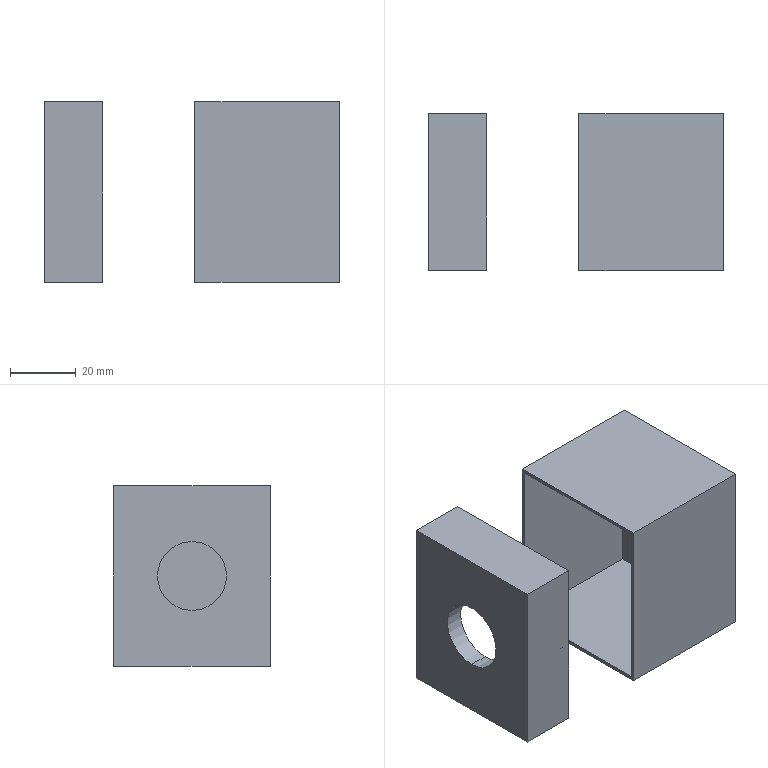Component | SolidWorks | BearingHousing-1 | 2 solids | 29 faces | box 89.77 x 47.79 x 55 mm | volume 29257 mm3 | plane 24 | cylinder 5 | commonest cylinder face diameters 47.04 x3 21 x2
STEP:
#1=COLOUR_RGB('',0.7922,0.8196,0.9333);
#2=FILL_AREA_STYLE_COLOUR('',#1);
#3=FILL_AREA_STYLE('',(#2));
#4=SURFACE_STYLE_FILL_AREA(#3);
#5=SURFACE_SIDE_STYLE('',(#4));
#6=SURFACE_STYLE_USAGE(.BOTH.,#5);
#7=PRESENTATION_STYLE_ASSIGNMENT((#6));
#8=CARTESIAN_POINT('',(7.039,3.272,1.043));
#9=VERTEX_POINT('',#8);
#10=CARTESIAN_POINT('',(7.039,1.469,1.043));
#11=VERTEX_POINT('',#10);
#12=CARTESIAN_POINT('',(7.039,3.37,1.043));
#13=DIRECTION('',(0.,-1.,0.));
#14=VECTOR('',#13,39.37);
#15=LINE('',#12,#14);
#16=EDGE_CURVE('',#9,#11,#15,.T.);
#17=ORIENTED_EDGE('',*,*,#16,.T.);
#18=CARTESIAN_POINT('',(7.039,1.469,-1.043));
#19=VERTEX_POINT('',#18);
#20=CARTESIAN_POINT('',(7.039,1.469,0.8331));
#21=DIRECTION('',(-0.,-0.,-1.));
#22=VECTOR('',#21,39.37);
#23=LINE('',#20,#22);
#24=EDGE_CURVE('',#11,#19,#23,.T.);
#25=ORIENTED_EDGE('',*,*,#24,.T.);
#26=CARTESIAN_POINT('',(7.039,3.272,-1.043));
#27=VERTEX_POINT('',#26);
#28=CARTESIAN_POINT('',(7.039,3.37,-1.043));
#29=DIRECTION('',(-0.,1.,-0.));
#30=VECTOR('',#29,39.37);
#31=LINE('',#28,#30);
#32=EDGE_CURVE('',#19,#27,#31,.T.);
#33=ORIENTED_EDGE('',*,*,#32,.T.);
#34=CARTESIAN_POINT('',(7.039,3.272,0.8331));
#35=DIRECTION('',(0.,0.,1.));
#36=VECTOR('',#35,39.37);
#37=LINE('',#34,#36);
#38=EDGE_CURVE('',#27,#9,#37,.T.);
#39=ORIENTED_EDGE('',*,*,#38,.T.);
#40=EDGE_LOOP('',(#17,#25,#33,#39));
#41=FACE_BOUND('',#40,.T.);
#42=CARTESIAN_POINT('',(7.039,1.43,1.083));
#43=VERTEX_POINT('',#42);
#44=CARTESIAN_POINT('',(7.039,1.43,-1.083));
#45=VERTEX_POINT('',#44);
#46=CARTESIAN_POINT('',(7.039,1.43,1.083));
#47=DIRECTION('',(-0.,-0.,-1.));
#48=VECTOR('',#47,39.37);
#49=LINE('',#46,#48);
#50=EDGE_CURVE('',#43,#45,#49,.T.);
#51=ORIENTED_EDGE('',*,*,#50,.F.);
#52=CARTESIAN_POINT('',(7.039,3.312,1.083));
#53=VERTEX_POINT('',#52);
#54=CARTESIAN_POINT('',(7.039,3.312,1.083));
#55=DIRECTION('',(0.,-1.,0.));
#56=VECTOR('',#55,39.37);
#57=LINE('',#54,#56);
#58=EDGE_CURVE('',#53,#43,#57,.T.);
#59=ORIENTED_EDGE('',*,*,#58,.F.);
#60=CARTESIAN_POINT('',(7.039,3.312,-1.083));
#61=VERTEX_POINT('',#60);
#62=CARTESIAN_POINT('',(7.039,3.312,-1.083));
#63=DIRECTION('',(0.,0.,1.));
#64=VECTOR('',#63,39.37);
#65=LINE('',#62,#64);
#66=EDGE_CURVE('',#61,#53,#65,.T.);
#67=ORIENTED_EDGE('',*,*,#66,.F.);
#68=CARTESIAN_POINT('',(7.039,1.43,-1.083));
#69=DIRECTION('',(-0.,1.,-0.));
#70=VECTOR('',#69,39.37);
#71=LINE('',#68,#70);
#72=EDGE_CURVE('',#45,#61,#71,.T.);
#73=ORIENTED_EDGE('',*,*,#72,.F.);
#74=EDGE_LOOP('',(#51,#59,#67,#73));
#75=FACE_OUTER_BOUND('',#74,.T.);
#76=CARTESIAN_POINT('',(7.039,3.37,0.8331));
#77=DIRECTION('',(1.,0.,-0.));
#78=DIRECTION('',(0.,-1.,0.));
#79=AXIS2_PLACEMENT_3D('',#76,#77,#78);
#80=PLANE('',#79);
#81=ADVANCED_FACE('',(#41,#75),#80,.F.);
#82=CARTESIAN_POINT('',(8.771,1.43,-1.083));
#83=VERTEX_POINT('',#82);
#84=CARTESIAN_POINT('',(-2.164,1.43,-1.083));
#85=DIRECTION('',(1.,-0.,0.));
#86=VECTOR('',#85,39.37);
#87=LINE('',#84,#86);
#88=EDGE_CURVE('',#45,#83,#87,.T.);
#89=ORIENTED_EDGE('',*,*,#88,.F.);
#90=ORIENTED_EDGE('',*,*,#72,.T.);
#91=CARTESIAN_POINT('',(8.771,3.312,-1.083));
#92=VERTEX_POINT('',#91);
#93=CARTESIAN_POINT('',(-2.164,3.312,-1.083));
#94=DIRECTION('',(-1.,-0.,-0.));
#95=VECTOR('',#94,39.37);
#96=LINE('',#93,#95);
#97=EDGE_CURVE('',#92,#61,#96,.T.);
#98=ORIENTED_EDGE('',*,*,#97,.F.);
#99=CARTESIAN_POINT('',(8.771,1.43,-1.083));
#100=DIRECTION('',(-0.,1.,-0.));
#101=VECTOR('',#100,39.37);
#102=LINE('',#99,#101);
#103=EDGE_CURVE('',#83,#92,#102,.T.);
#104=ORIENTED_EDGE('',*,*,#103,.F.);
#105=EDGE_LOOP('',(#89,#90,#98,#104));
#106=FACE_OUTER_BOUND('',#105,.T.);
#107=CARTESIAN_POINT('',(-2.164,3.37,-1.083));
#108=DIRECTION('',(-0.,0.,1.));
#109=DIRECTION('',(0.,-1.,0.));
#110=AXIS2_PLACEMENT_3D('',#107,#108,#109);
#111=PLANE('',#110);
#112=ADVANCED_FACE('',(#106),#111,.F.);
#113=ORIENTED_EDGE('',*,*,#58,.T.);
#114=CARTESIAN_POINT('',(8.771,1.43,1.083));
#115=VERTEX_POINT('',#114);
#116=CARTESIAN_POINT('',(-2.164,1.43,1.083));
#117=DIRECTION('',(1.,-0.,0.));
#118=VECTOR('',#117,39.37);
#119=LINE('',#116,#118);
#120=EDGE_CURVE('',#43,#115,#119,.T.);
#121=ORIENTED_EDGE('',*,*,#120,.T.);
#122=CARTESIAN_POINT('',(8.771,3.312,1.083));
#123=VERTEX_POINT('',#122);
#124=CARTESIAN_POINT('',(8.771,3.312,1.083));
#125=DIRECTION('',(0.,-1.,0.));
#126=VECTOR('',#125,39.37);
#127=LINE('',#124,#126);
#128=EDGE_CURVE('',#123,#115,#127,.T.);
#129=ORIENTED_EDGE('',*,*,#128,.F.);
#130=CARTESIAN_POINT('',(-2.164,3.312,1.083));
#131=DIRECTION('',(-1.,-0.,-0.));
#132=VECTOR('',#131,39.37);
#133=LINE('',#130,#132);
#134=EDGE_CURVE('',#123,#53,#133,.T.);
#135=ORIENTED_EDGE('',*,*,#134,.T.);
#136=EDGE_LOOP('',(#113,#121,#129,#135));
#137=FACE_OUTER_BOUND('',#136,.T.);
#138=CARTESIAN_POINT('',(-2.164,3.37,1.083));
#139=DIRECTION('',(-0.,0.,1.));
#140=DIRECTION('',(0.,-1.,0.));
#141=AXIS2_PLACEMENT_3D('',#138,#139,#140);
#142=PLANE('',#141);
#143=ADVANCED_FACE('',(#137),#142,.T.);
#144=ORIENTED_EDGE('',*,*,#120,.F.);
#145=ORIENTED_EDGE('',*,*,#50,.T.);
#146=ORIENTED_EDGE('',*,*,#88,.T.);
#147=CARTESIAN_POINT('',(8.771,1.43,1.083));
#148=DIRECTION('',(-0.,-0.,-1.));
#149=VECTOR('',#148,39.37);
#150=LINE('',#147,#149);
#151=EDGE_CURVE('',#115,#83,#150,.T.);
#152=ORIENTED_EDGE('',*,*,#151,.F.);
#153=EDGE_LOOP('',(#144,#145,#146,#152));
#154=FACE_OUTER_BOUND('',#153,.T.);
#155=CARTESIAN_POINT('',(-2.164,1.43,1.083));
#156=DIRECTION('',(0.,1.,-0.));
#157=DIRECTION('',(0.,0.,1.));
#158=AXIS2_PLACEMENT_3D('',#155,#156,#157);
#159=PLANE('',#158);
#160=ADVANCED_FACE('',(#154),#159,.F.);
#161=ORIENTED_EDGE('',*,*,#97,.T.);
#162=ORIENTED_EDGE('',*,*,#66,.T.);
#163=ORIENTED_EDGE('',*,*,#134,.F.);
#164=CARTESIAN_POINT('',(8.771,3.312,-1.083));
#165=DIRECTION('',(0.,0.,1.));
#166=VECTOR('',#165,39.37);
#167=LINE('',#164,#166);
#168=EDGE_CURVE('',#92,#123,#167,.T.);
#169=ORIENTED_EDGE('',*,*,#168,.F.);
#170=EDGE_LOOP('',(#161,#162,#163,#169));
#171=FACE_OUTER_BOUND('',#170,.T.);
#172=CARTESIAN_POINT('',(-2.164,3.312,1.083));
#173=DIRECTION('',(0.,-1.,0.));
#174=DIRECTION('',(-0.,-0.,-1.));
#175=AXIS2_PLACEMENT_3D('',#172,#173,#174);
#176=PLANE('',#175);
#177=ADVANCED_FACE('',(#171),#176,.F.);
#178=CARTESIAN_POINT('',(8.692,1.469,1.043));
#179=VERTEX_POINT('',#178);
#180=CARTESIAN_POINT('',(8.692,1.469,-1.043));
#181=VERTEX_POINT('',#180);
#182=CARTESIAN_POINT('',(8.692,1.469,1.043));
#183=DIRECTION('',(-0.,-0.,-1.));
#184=VECTOR('',#183,39.37);
#185=LINE('',#182,#184);
#186=EDGE_CURVE('',#179,#181,#185,.T.);
#187=ORIENTED_EDGE('',*,*,#186,.T.);
#188=CARTESIAN_POINT('',(5.464,1.469,-1.043));
#189=DIRECTION('',(1.,0.,0.));
#190=VECTOR('',#189,39.37);
#191=LINE('',#188,#190);
#192=EDGE_CURVE('',#19,#181,#191,.T.);
#193=ORIENTED_EDGE('',*,*,#192,.F.);
#194=ORIENTED_EDGE('',*,*,#24,.F.);
#195=CARTESIAN_POINT('',(5.464,1.469,1.043));
#196=DIRECTION('',(1.,0.,0.));
#197=VECTOR('',#196,39.37);
#198=LINE('',#195,#197);
#199=EDGE_CURVE('',#11,#179,#198,.T.);
#200=ORIENTED_EDGE('',*,*,#199,.T.);
#201=EDGE_LOOP('',(#187,#193,#194,#200));
#202=FACE_OUTER_BOUND('',#201,.T.);
#203=CARTESIAN_POINT('',(5.464,1.469,1.043));
#204=DIRECTION('',(0.,-1.,0.));
#205=DIRECTION('',(-0.,-0.,-1.));
#206=AXIS2_PLACEMENT_3D('',#203,#204,#205);
#207=PLANE('',#206);
#208=ADVANCED_FACE('',(#202),#207,.F.);
#209=CARTESIAN_POINT('',(8.692,3.272,1.043));
#210=VERTEX_POINT('',#209);
#211=CARTESIAN_POINT('',(8.692,3.272,1.043));
#212=DIRECTION('',(0.,-1.,0.));
#213=VECTOR('',#212,39.37);
#214=LINE('',#211,#213);
#215=EDGE_CURVE('',#210,#179,#214,.T.);
#216=ORIENTED_EDGE('',*,*,#215,.T.);
#217=ORIENTED_EDGE('',*,*,#199,.F.);
#218=ORIENTED_EDGE('',*,*,#16,.F.);
#219=CARTESIAN_POINT('',(5.464,3.272,1.043));
#220=DIRECTION('',(1.,0.,0.));
#221=VECTOR('',#220,39.37);
#222=LINE('',#219,#221);
#223=EDGE_CURVE('',#9,#210,#222,.T.);
#224=ORIENTED_EDGE('',*,*,#223,.T.);
#225=EDGE_LOOP('',(#216,#217,#218,#224));
#226=FACE_OUTER_BOUND('',#225,.T.);
#227=CARTESIAN_POINT('',(5.464,3.272,1.043));
#228=DIRECTION('',(-0.,0.,1.));
#229=DIRECTION('',(0.,-1.,0.));
#230=AXIS2_PLACEMENT_3D('',#227,#228,#229);
#231=PLANE('',#230);
#232=ADVANCED_FACE('',(#226),#231,.F.);
#233=CARTESIAN_POINT('',(8.692,3.272,-1.043));
#234=VERTEX_POINT('',#233);
#235=CARTESIAN_POINT('',(8.692,3.272,-1.043));
#236=DIRECTION('',(0.,0.,1.));
#237=VECTOR('',#236,39.37);
#238=LINE('',#235,#237);
#239=EDGE_CURVE('',#234,#210,#238,.T.);
#240=ORIENTED_EDGE('',*,*,#239,.T.);
#241=ORIENTED_EDGE('',*,*,#223,.F.);
#242=ORIENTED_EDGE('',*,*,#38,.F.);
#243=CARTESIAN_POINT('',(5.464,3.272,-1.043));
#244=DIRECTION('',(1.,0.,0.));
#245=VECTOR('',#244,39.37);
#246=LINE('',#243,#245);
#247=EDGE_CURVE('',#27,#234,#246,.T.);
#248=ORIENTED_EDGE('',*,*,#247,.T.);
#249=EDGE_LOOP('',(#240,#241,#242,#248));
#250=FACE_OUTER_BOUND('',#249,.T.);
#251=CARTESIAN_POINT('',(5.464,3.272,-1.043));
#252=DIRECTION('',(-0.,1.,-0.));
#253=DIRECTION('',(0.,0.,1.));
#254=AXIS2_PLACEMENT_3D('',#251,#252,#253);
#255=PLANE('',#254);
#256=ADVANCED_FACE('',(#250),#255,.F.);
#257=CARTESIAN_POINT('',(8.692,1.469,-1.043));
#258=DIRECTION('',(-0.,1.,-0.));
#259=VECTOR('',#258,39.37);
#260=LINE('',#257,#259);
#261=EDGE_CURVE('',#181,#234,#260,.T.);
#262=ORIENTED_EDGE('',*,*,#261,.T.);
#263=ORIENTED_EDGE('',*,*,#247,.F.);
#264=ORIENTED_EDGE('',*,*,#32,.F.);
#265=ORIENTED_EDGE('',*,*,#192,.T.);
#266=EDGE_LOOP('',(#262,#263,#264,#265));
#267=FACE_OUTER_BOUND('',#266,.T.);
#268=CARTESIAN_POINT('',(5.464,1.469,-1.043));
#269=DIRECTION('',(0.,-0.,-1.));
#270=DIRECTION('',(-0.,1.,-0.));
#271=AXIS2_PLACEMENT_3D('',#268,#269,#270);
#272=PLANE('',#271);
#273=ADVANCED_FACE('',(#267),#272,.F.);
#274=ORIENTED_EDGE('',*,*,#151,.T.);
#275=ORIENTED_EDGE('',*,*,#103,.T.);
#276=ORIENTED_EDGE('',*,*,#168,.T.);
#277=ORIENTED_EDGE('',*,*,#128,.T.);
#278=EDGE_LOOP('',(#274,#275,#276,#277));
#279=FACE_OUTER_BOUND('',#278,.T.);
#280=CARTESIAN_POINT('',(8.771,3.37,0.8331));
#281=DIRECTION('',(1.,0.,-0.));
#282=DIRECTION('',(0.,-1.,0.));
#283=AXIS2_PLACEMENT_3D('',#280,#281,#282);
#284=PLANE('',#283);
#285=ADVANCED_FACE('',(#279),#284,.T.);
#286=ORIENTED_EDGE('',*,*,#215,.F.);
#287=ORIENTED_EDGE('',*,*,#239,.F.);
#288=ORIENTED_EDGE('',*,*,#261,.F.);
#289=ORIENTED_EDGE('',*,*,#186,.F.);
#290=EDGE_LOOP('',(#286,#287,#288,#289));
#291=FACE_OUTER_BOUND('',#290,.T.);
#292=CARTESIAN_POINT('',(8.692,3.37,0.8331));
#293=DIRECTION('',(1.,0.,-0.));
#294=DIRECTION('',(0.,-1.,0.));
#295=AXIS2_PLACEMENT_3D('',#292,#293,#294);
#296=PLANE('',#295);
#297=ADVANCED_FACE('',(#291),#296,.F.);
#298=CLOSED_SHELL('',(#81,#112,#143,#160,#177,#208,#232,#256,#273,#285,#297));
#299=MANIFOLD_SOLID_BREP('',#298);
#300=STYLED_ITEM('',(#7),#299);
#301=(LENGTH_UNIT()NAMED_UNIT(*)SI_UNIT($,.METRE.));
#302=LENGTH_MEASURE_WITH_UNIT(LENGTH_MEASURE(0.0254),#301);
#303=DIMENSIONAL_EXPONENTS(1.,0.,0.,0.,0.,0.,0.);
#304=(CONVERSION_BASED_UNIT('',#302)LENGTH_UNIT()NAMED_UNIT(#303));
#305=UNCERTAINTY_MEASURE_WITH_UNIT(LENGTH_MEASURE(0.00001),#304,'','');
#306=(NAMED_UNIT(*)PLANE_ANGLE_UNIT()SI_UNIT($,.RADIAN.));
#307=(NAMED_UNIT(*)SI_UNIT($,.STERADIAN.)SOLID_ANGLE_UNIT());
#308=(GEOMETRIC_REPRESENTATION_CONTEXT(3)GLOBAL_UNCERTAINTY_ASSIGNED_CONTEXT((#305))GLOBAL_UNIT_ASSIGNED_CONTEXT((#304,#306,#307))REPRESENTATION_CONTEXT('',''));
#309=MECHANICAL_DESIGN_GEOMETRIC_PRESENTATION_REPRESENTATION('',(#300),#308);
#310=COLOUR_RGB('',0.7922,0.8196,0.9333);
#311=FILL_AREA_STYLE_COLOUR('',#310);
#312=FILL_AREA_STYLE('',(#311));
#313=SURFACE_STYLE_FILL_AREA(#312);
#314=SURFACE_SIDE_STYLE('',(#313));
#315=SURFACE_STYLE_USAGE(.BOTH.,#314);
#316=PRESENTATION_STYLE_ASSIGNMENT((#315));
#317=CARTESIAN_POINT('',(5.752,1.445,0.));
#318=VERTEX_POINT('',#317);
#319=CARTESIAN_POINT('',(5.752,1.469,-0.212));
#320=VERTEX_POINT('',#319);
#321=CARTESIAN_POINT('',(5.752,2.371,0.));
#322=DIRECTION('',(1.,0.,-0.));
#323=DIRECTION('',(0.,-1.,0.));
#324=AXIS2_PLACEMENT_3D('',#321,#322,#323);
#325=CIRCLE('',#324,0.926);
#326=EDGE_CURVE('',#318,#320,#325,.T.);
#327=ORIENTED_EDGE('',*,*,#326,.F.);
#328=CARTESIAN_POINT('',(5.936,1.445,0.));
#329=VERTEX_POINT('',#328);
#330=CARTESIAN_POINT('',(5.752,1.445,0.));
#331=DIRECTION('',(1.,0.,-0.));
#332=VECTOR('',#331,39.37);
#333=LINE('',#330,#332);
#334=EDGE_CURVE('',#318,#329,#333,.T.);
#335=ORIENTED_EDGE('',*,*,#334,.T.);
#336=CARTESIAN_POINT('',(5.936,1.469,-0.212));
#337=VERTEX_POINT('',#336);
#338=CARTESIAN_POINT('',(5.936,2.371,0.));
#339=DIRECTION('',(1.,0.,-0.));
#340=DIRECTION('',(0.,-1.,0.));
#341=AXIS2_PLACEMENT_3D('',#338,#339,#340);
#342=CIRCLE('',#341,0.926);
#343=EDGE_CURVE('',#329,#337,#342,.T.);
#344=ORIENTED_EDGE('',*,*,#343,.T.);
#345=CARTESIAN_POINT('',(5.752,1.469,-0.212));
#346=DIRECTION('',(1.,0.,-0.));
#347=VECTOR('',#346,39.37);
#348=LINE('',#345,#347);
#349=EDGE_CURVE('',#320,#337,#348,.T.);
#350=ORIENTED_EDGE('',*,*,#349,.F.);
#351=EDGE_LOOP('',(#327,#335,#344,#350));
#352=FACE_OUTER_BOUND('',#351,.T.);
#353=CARTESIAN_POINT('',(5.752,2.371,0.));
#354=DIRECTION('',(1.,0.,-0.));
#355=DIRECTION('',(0.,-1.,0.));
#356=AXIS2_PLACEMENT_3D('',#353,#354,#355);
#357=CYLINDRICAL_SURFACE('',#356,0.926);
#358=ADVANCED_FACE('',(#352),#357,.F.);
#359=CARTESIAN_POINT('',(5.464,2.371,-0.4134));
#360=VERTEX_POINT('',#359);
#361=CARTESIAN_POINT('',(5.464,2.371,0.4134));
#362=VERTEX_POINT('',#361);
#363=CARTESIAN_POINT('',(5.464,2.371,-0.));
#364=DIRECTION('',(-1.,-0.,0.));
#365=DIRECTION('',(0.,-1.,0.));
#366=AXIS2_PLACEMENT_3D('',#363,#364,#365);
#367=CIRCLE('',#366,0.4134);
#368=EDGE_CURVE('',#360,#362,#367,.T.);
#369=ORIENTED_EDGE('',*,*,#368,.F.);
#370=CARTESIAN_POINT('',(5.237,2.371,-0.4134));
#371=VERTEX_POINT('',#370);
#372=CARTESIAN_POINT('',(7.639,2.371,-0.4134));
#373=DIRECTION('',(-1.,-0.,-0.));
#374=VECTOR('',#373,39.37);
#375=LINE('',#372,#374);
#376=EDGE_CURVE('',#360,#371,#375,.T.);
#377=ORIENTED_EDGE('',*,*,#376,.T.);
#378=CARTESIAN_POINT('',(5.237,2.371,0.4134));
#379=VERTEX_POINT('',#378);
#380=CARTESIAN_POINT('',(5.237,2.371,-0.));
#381=DIRECTION('',(-1.,-0.,-0.));
#382=DIRECTION('',(0.,0.,1.));
#383=AXIS2_PLACEMENT_3D('',#380,#381,#382);
#384=CIRCLE('',#383,0.4134);
#385=EDGE_CURVE('',#371,#379,#384,.T.);
#386=ORIENTED_EDGE('',*,*,#385,.T.);
#387=CARTESIAN_POINT('',(7.639,2.371,0.4134));
#388=DIRECTION('',(-1.,-0.,-0.));
#389=VECTOR('',#388,39.37);
#390=LINE('',#387,#389);
#391=EDGE_CURVE('',#362,#379,#390,.T.);
#392=ORIENTED_EDGE('',*,*,#391,.F.);
#393=EDGE_LOOP('',(#369,#377,#386,#392));
#394=FACE_OUTER_BOUND('',#393,.T.);
#395=CARTESIAN_POINT('',(7.639,2.371,0.));
#396=DIRECTION('',(-1.,-0.,-0.));
#397=DIRECTION('',(0.,0.,1.));
#398=AXIS2_PLACEMENT_3D('',#395,#396,#397);
#399=CYLINDRICAL_SURFACE('',#398,0.4134);
#400=ADVANCED_FACE('',(#394),#399,.F.);
#401=CARTESIAN_POINT('',(5.237,1.43,1.083));
#402=VERTEX_POINT('',#401);
#403=CARTESIAN_POINT('',(5.936,1.43,1.083));
#404=VERTEX_POINT('',#403);
#405=CARTESIAN_POINT('',(-2.164,1.43,1.083));
#406=DIRECTION('',(1.,-0.,0.));
#407=VECTOR('',#406,39.37);
#408=LINE('',#405,#407);
#409=EDGE_CURVE('',#402,#404,#408,.T.);
#410=ORIENTED_EDGE('',*,*,#409,.T.);
#411=CARTESIAN_POINT('',(5.936,3.312,1.083));
#412=VERTEX_POINT('',#411);
#413=CARTESIAN_POINT('',(5.936,3.312,1.083));
#414=DIRECTION('',(0.,-1.,0.));
#415=VECTOR('',#414,39.37);
#416=LINE('',#413,#415);
#417=EDGE_CURVE('',#412,#404,#416,.T.);
#418=ORIENTED_EDGE('',*,*,#417,.F.);
#419=CARTESIAN_POINT('',(5.237,3.312,1.083));
#420=VERTEX_POINT('',#419);
#421=CARTESIAN_POINT('',(-2.164,3.312,1.083));
#422=DIRECTION('',(-1.,-0.,-0.));
#423=VECTOR('',#422,39.37);
#424=LINE('',#421,#423);
#425=EDGE_CURVE('',#412,#420,#424,.T.);
#426=ORIENTED_EDGE('',*,*,#425,.T.);
#427=CARTESIAN_POINT('',(5.237,3.37,1.083));
#428=DIRECTION('',(0.,-1.,0.));
#429=VECTOR('',#428,39.37);
#430=LINE('',#427,#429);
#431=EDGE_CURVE('',#420,#402,#430,.T.);
#432=ORIENTED_EDGE('',*,*,#431,.T.);
#433=EDGE_LOOP('',(#410,#418,#426,#432));
#434=FACE_OUTER_BOUND('',#433,.T.);
#435=CARTESIAN_POINT('',(-2.164,3.37,1.083));
#436=DIRECTION('',(-0.,0.,1.));
#437=DIRECTION('',(0.,-1.,0.));
#438=AXIS2_PLACEMENT_3D('',#435,#436,#437);
#439=PLANE('',#438);
#440=ADVANCED_FACE('',(#434),#439,.T.);
#441=CARTESIAN_POINT('',(5.936,3.312,-1.083));
#442=VERTEX_POINT('',#441);
#443=CARTESIAN_POINT('',(5.936,3.312,-1.083));
#444=DIRECTION('',(0.,0.,1.));
#445=VECTOR('',#444,39.37);
#446=LINE('',#443,#445);
#447=EDGE_CURVE('',#442,#412,#446,.T.);
#448=ORIENTED_EDGE('',*,*,#447,.F.);
#449=CARTESIAN_POINT('',(5.237,3.312,-1.083));
#450=VERTEX_POINT('',#449);
#451=CARTESIAN_POINT('',(-2.164,3.312,-1.083));
#452=DIRECTION('',(-1.,-0.,-0.));
#453=VECTOR('',#452,39.37);
#454=LINE('',#451,#453);
#455=EDGE_CURVE('',#442,#450,#454,.T.);
#456=ORIENTED_EDGE('',*,*,#455,.T.);
#457=CARTESIAN_POINT('',(5.237,3.312,1.083));
#458=DIRECTION('',(0.,-0.,-1.));
#459=VECTOR('',#458,39.37);
#460=LINE('',#457,#459);
#461=EDGE_CURVE('',#420,#450,#460,.T.);
#462=ORIENTED_EDGE('',*,*,#461,.F.);
#463=ORIENTED_EDGE('',*,*,#425,.F.);
#464=EDGE_LOOP('',(#448,#456,#462,#463));
#465=FACE_OUTER_BOUND('',#464,.T.);
#466=CARTESIAN_POINT('',(-2.164,3.312,1.083));
#467=DIRECTION('',(0.,-1.,0.));
#468=DIRECTION('',(-0.,-0.,-1.));
#469=AXIS2_PLACEMENT_3D('',#466,#467,#468);
#470=PLANE('',#469);
#471=ADVANCED_FACE('',(#465),#470,.F.);
#472=CARTESIAN_POINT('',(5.936,1.43,-1.083));
#473=VERTEX_POINT('',#472);
#474=CARTESIAN_POINT('',(5.936,1.43,-1.083));
#475=DIRECTION('',(-0.,1.,-0.));
#476=VECTOR('',#475,39.37);
#477=LINE('',#474,#476);
#478=EDGE_CURVE('',#473,#442,#477,.T.);
#479=ORIENTED_EDGE('',*,*,#478,.F.);
#480=CARTESIAN_POINT('',(5.237,1.43,-1.083));
#481=VERTEX_POINT('',#480);
#482=CARTESIAN_POINT('',(-2.164,1.43,-1.083));
#483=DIRECTION('',(1.,-0.,0.));
#484=VECTOR('',#483,39.37);
#485=LINE('',#482,#484);
#486=EDGE_CURVE('',#481,#473,#485,.T.);
#487=ORIENTED_EDGE('',*,*,#486,.F.);
#488=CARTESIAN_POINT('',(5.237,3.37,-1.083));
#489=DIRECTION('',(0.,-1.,0.));
#490=VECTOR('',#489,39.37);
#491=LINE('',#488,#490);
#492=EDGE_CURVE('',#450,#481,#491,.T.);
#493=ORIENTED_EDGE('',*,*,#492,.F.);
#494=ORIENTED_EDGE('',*,*,#455,.F.);
#495=EDGE_LOOP('',(#479,#487,#493,#494));
#496=FACE_OUTER_BOUND('',#495,.T.);
#497=CARTESIAN_POINT('',(-2.164,3.37,-1.083));
#498=DIRECTION('',(-0.,0.,1.));
#499=DIRECTION('',(0.,-1.,0.));
#500=AXIS2_PLACEMENT_3D('',#497,#498,#499);
#501=PLANE('',#500);
#502=ADVANCED_FACE('',(#496),#501,.F.);
#503=CARTESIAN_POINT('',(5.237,2.371,-0.));
#504=DIRECTION('',(-1.,-0.,-0.));
#505=DIRECTION('',(0.,0.,1.));
#506=AXIS2_PLACEMENT_3D('',#503,#504,#505);
#507=CIRCLE('',#506,0.4134);
#508=EDGE_CURVE('',#379,#371,#507,.T.);
#509=ORIENTED_EDGE('',*,*,#508,.F.);
#510=ORIENTED_EDGE('',*,*,#385,.F.);
#511=EDGE_LOOP('',(#509,#510));
#512=FACE_BOUND('',#511,.T.);
#513=ORIENTED_EDGE('',*,*,#492,.T.);
#514=CARTESIAN_POINT('',(5.237,1.43,1.083));
#515=DIRECTION('',(0.,-0.,-1.));
#516=VECTOR('',#515,39.37);
#517=LINE('',#514,#516);
#518=EDGE_CURVE('',#402,#481,#517,.T.);
#519=ORIENTED_EDGE('',*,*,#518,.F.);
#520=ORIENTED_EDGE('',*,*,#431,.F.);
#521=ORIENTED_EDGE('',*,*,#461,.T.);
#522=EDGE_LOOP('',(#513,#519,#520,#521));
#523=FACE_OUTER_BOUND('',#522,.T.);
#524=CARTESIAN_POINT('',(5.237,3.37,1.083));
#525=DIRECTION('',(1.,0.,0.));
#526=DIRECTION('',(0.,-0.,-1.));
#527=AXIS2_PLACEMENT_3D('',#524,#525,#526);
#528=PLANE('',#527);
#529=ADVANCED_FACE('',(#512,#523),#528,.F.);
#530=ORIENTED_EDGE('',*,*,#376,.F.);
#531=CARTESIAN_POINT('',(5.464,2.371,-0.));
#532=DIRECTION('',(-1.,-0.,0.));
#533=DIRECTION('',(0.,-1.,0.));
#534=AXIS2_PLACEMENT_3D('',#531,#532,#533);
#535=CIRCLE('',#534,0.4134);
#536=EDGE_CURVE('',#362,#360,#535,.T.);
#537=ORIENTED_EDGE('',*,*,#536,.F.);
#538=ORIENTED_EDGE('',*,*,#391,.T.);
#539=ORIENTED_EDGE('',*,*,#508,.T.);
#540=EDGE_LOOP('',(#530,#537,#538,#539));
#541=FACE_OUTER_BOUND('',#540,.T.);
#542=CARTESIAN_POINT('',(7.639,2.371,0.));
#543=DIRECTION('',(-1.,-0.,-0.));
#544=DIRECTION('',(0.,0.,1.));
#545=AXIS2_PLACEMENT_3D('',#542,#543,#544);
#546=CYLINDRICAL_SURFACE('',#545,0.4134);
#547=ADVANCED_FACE('',(#541),#546,.F.);
#548=CARTESIAN_POINT('',(5.936,1.43,1.083));
#549=DIRECTION('',(-0.,-0.,-1.));
#550=VECTOR('',#549,39.37);
#551=LINE('',#548,#550);
#552=EDGE_CURVE('',#404,#473,#551,.T.);
#553=ORIENTED_EDGE('',*,*,#552,.F.);
#554=ORIENTED_EDGE('',*,*,#409,.F.);
#555=ORIENTED_EDGE('',*,*,#518,.T.);
#556=ORIENTED_EDGE('',*,*,#486,.T.);
#557=EDGE_LOOP('',(#553,#554,#555,#556));
#558=FACE_OUTER_BOUND('',#557,.T.);
#559=CARTESIAN_POINT('',(-2.164,1.43,1.083));
#560=DIRECTION('',(0.,1.,-0.));
#561=DIRECTION('',(0.,0.,1.));
#562=AXIS2_PLACEMENT_3D('',#559,#560,#561);
#563=PLANE('',#562);
#564=ADVANCED_FACE('',(#558),#563,.F.);
#565=CARTESIAN_POINT('',(5.936,3.272,-0.212));
#566=VERTEX_POINT('',#565);
#567=CARTESIAN_POINT('',(5.936,3.272,0.212));
#568=VERTEX_POINT('',#567);
#569=CARTESIAN_POINT('',(5.936,2.371,0.));
#570=DIRECTION('',(1.,0.,-0.));
#571=DIRECTION('',(0.,-1.,0.));
#572=AXIS2_PLACEMENT_3D('',#569,#570,#571);
#573=CIRCLE('',#572,0.926);
#574=EDGE_CURVE('',#566,#568,#573,.T.);
#575=ORIENTED_EDGE('',*,*,#574,.F.);
#576=CARTESIAN_POINT('',(5.936,3.272,-1.043));
#577=VERTEX_POINT('',#576);
#578=CARTESIAN_POINT('',(5.936,3.272,0.8331));
#579=DIRECTION('',(0.,0.,1.));
#580=VECTOR('',#579,39.37);
#581=LINE('',#578,#580);
#582=EDGE_CURVE('',#577,#566,#581,.T.);
#583=ORIENTED_EDGE('',*,*,#582,.F.);
#584=CARTESIAN_POINT('',(5.936,1.469,-1.043));
#585=VERTEX_POINT('',#584);
#586=CARTESIAN_POINT('',(5.936,3.37,-1.043));
#587=DIRECTION('',(-0.,1.,-0.));
#588=VECTOR('',#587,39.37);
#589=LINE('',#586,#588);
#590=EDGE_CURVE('',#585,#577,#589,.T.);
#591=ORIENTED_EDGE('',*,*,#590,.F.);
#592=CARTESIAN_POINT('',(5.936,1.469,0.8331));
#593=DIRECTION('',(-0.,-0.,-1.));
#594=VECTOR('',#593,39.37);
#595=LINE('',#592,#594);
#596=EDGE_CURVE('',#337,#585,#595,.T.);
#597=ORIENTED_EDGE('',*,*,#596,.F.);
#598=ORIENTED_EDGE('',*,*,#343,.F.);
#599=CARTESIAN_POINT('',(5.936,1.469,0.212));
#600=VERTEX_POINT('',#599);
#601=CARTESIAN_POINT('',(5.936,2.371,0.));
#602=DIRECTION('',(1.,0.,-0.));
#603=DIRECTION('',(0.,-1.,0.));
#604=AXIS2_PLACEMENT_3D('',#601,#602,#603);
#605=CIRCLE('',#604,0.926);
#606=EDGE_CURVE('',#600,#329,#605,.T.);
#607=ORIENTED_EDGE('',*,*,#606,.F.);
#608=CARTESIAN_POINT('',(5.936,1.469,1.043));
#609=VERTEX_POINT('',#608);
#610=CARTESIAN_POINT('',(5.936,1.469,0.8331));
#611=DIRECTION('',(-0.,-0.,-1.));
#612=VECTOR('',#611,39.37);
#613=LINE('',#610,#612);
#614=EDGE_CURVE('',#609,#600,#613,.T.);
#615=ORIENTED_EDGE('',*,*,#614,.F.);
#616=CARTESIAN_POINT('',(5.936,3.272,1.043));
#617=VERTEX_POINT('',#616);
#618=CARTESIAN_POINT('',(5.936,3.37,1.043));
#619=DIRECTION('',(0.,-1.,0.));
#620=VECTOR('',#619,39.37);
#621=LINE('',#618,#620);
#622=EDGE_CURVE('',#617,#609,#621,.T.);
#623=ORIENTED_EDGE('',*,*,#622,.F.);
#624=CARTESIAN_POINT('',(5.936,3.272,0.8331));
#625=DIRECTION('',(0.,0.,1.));
#626=VECTOR('',#625,39.37);
#627=LINE('',#624,#626);
#628=EDGE_CURVE('',#568,#617,#627,.T.);
#629=ORIENTED_EDGE('',*,*,#628,.F.);
#630=EDGE_LOOP('',(#575,#583,#591,#597,#598,#607,#615,#623,#629));
#631=FACE_BOUND('',#630,.T.);
#632=ORIENTED_EDGE('',*,*,#552,.T.);
#633=ORIENTED_EDGE('',*,*,#478,.T.);
#634=ORIENTED_EDGE('',*,*,#447,.T.);
#635=ORIENTED_EDGE('',*,*,#417,.T.);
#636=EDGE_LOOP('',(#632,#633,#634,#635));
#637=FACE_OUTER_BOUND('',#636,.T.);
#638=CARTESIAN_POINT('',(5.936,3.37,0.8331));
#639=DIRECTION('',(1.,0.,-0.));
#640=DIRECTION('',(0.,-1.,0.));
#641=AXIS2_PLACEMENT_3D('',#638,#639,#640);
#642=PLANE('',#641);
#643=ADVANCED_FACE('',(#631,#637),#642,.T.);
#644=CARTESIAN_POINT('',(5.464,1.469,1.043));
#645=VERTEX_POINT('',#644);
#646=CARTESIAN_POINT('',(5.464,1.469,-1.043));
#647=VERTEX_POINT('',#646);
#648=CARTESIAN_POINT('',(5.464,1.469,1.043));
#649=DIRECTION('',(-0.,-0.,-1.));
#650=VECTOR('',#649,39.37);
#651=LINE('',#648,#650);
#652=EDGE_CURVE('',#645,#647,#651,.T.);
#653=ORIENTED_EDGE('',*,*,#652,.T.);
#654=CARTESIAN_POINT('',(5.464,3.272,-1.043));
#655=VERTEX_POINT('',#654);
#656=CARTESIAN_POINT('',(5.464,1.469,-1.043));
#657=DIRECTION('',(-0.,1.,-0.));
#658=VECTOR('',#657,39.37);
#659=LINE('',#656,#658);
#660=EDGE_CURVE('',#647,#655,#659,.T.);
#661=ORIENTED_EDGE('',*,*,#660,.T.);
#662=CARTESIAN_POINT('',(5.464,3.272,1.043));
#663=VERTEX_POINT('',#662);
#664=CARTESIAN_POINT('',(5.464,3.272,-1.043));
#665=DIRECTION('',(0.,0.,1.));
#666=VECTOR('',#665,39.37);
#667=LINE('',#664,#666);
#668=EDGE_CURVE('',#655,#663,#667,.T.);
#669=ORIENTED_EDGE('',*,*,#668,.T.);
#670=CARTESIAN_POINT('',(5.464,3.272,1.043));
#671=DIRECTION('',(0.,-1.,0.));
#672=VECTOR('',#671,39.37);
#673=LINE('',#670,#672);
#674=EDGE_CURVE('',#663,#645,#673,.T.);
#675=ORIENTED_EDGE('',*,*,#674,.T.);
#676=EDGE_LOOP('',(#653,#661,#669,#675));
#677=FACE_OUTER_BOUND('',#676,.T.);
#678=ORIENTED_EDGE('',*,*,#536,.T.);
#679=ORIENTED_EDGE('',*,*,#368,.T.);
#680=EDGE_LOOP('',(#678,#679));
#681=FACE_BOUND('',#680,.T.);
#682=CARTESIAN_POINT('',(5.464,3.37,0.8331));
#683=DIRECTION('',(1.,0.,-0.));
#684=DIRECTION('',(0.,-1.,0.));
#685=AXIS2_PLACEMENT_3D('',#682,#683,#684);
#686=PLANE('',#685);
#687=ADVANCED_FACE('',(#677,#681),#686,.T.);
#688=ORIENTED_EDGE('',*,*,#590,.T.);
#689=CARTESIAN_POINT('',(5.464,3.272,-1.043));
#690=DIRECTION('',(1.,0.,0.));
#691=VECTOR('',#690,39.37);
#692=LINE('',#689,#691);
#693=EDGE_CURVE('',#655,#577,#692,.T.);
#694=ORIENTED_EDGE('',*,*,#693,.F.);
#695=ORIENTED_EDGE('',*,*,#660,.F.);
#696=CARTESIAN_POINT('',(5.464,1.469,-1.043));
#697=DIRECTION('',(1.,0.,0.));
#698=VECTOR('',#697,39.37);
#699=LINE('',#696,#698);
#700=EDGE_CURVE('',#647,#585,#699,.T.);
#701=ORIENTED_EDGE('',*,*,#700,.T.);
#702=EDGE_LOOP('',(#688,#694,#695,#701));
#703=FACE_OUTER_BOUND('',#702,.T.);
#704=CARTESIAN_POINT('',(5.464,1.469,-1.043));
#705=DIRECTION('',(0.,-0.,-1.));
#706=DIRECTION('',(-0.,1.,-0.));
#707=AXIS2_PLACEMENT_3D('',#704,#705,#706);
#708=PLANE('',#707);
#709=ADVANCED_FACE('',(#703),#708,.F.);
#710=CARTESIAN_POINT('',(5.752,3.272,0.212));
#711=VERTEX_POINT('',#710);
#712=CARTESIAN_POINT('',(5.752,3.272,-0.212));
#713=VERTEX_POINT('',#712);
#714=CARTESIAN_POINT('',(5.752,3.272,-1.043));
#715=DIRECTION('',(-0.,-0.,-1.));
#716=VECTOR('',#715,39.37);
#717=LINE('',#714,#716);
#718=EDGE_CURVE('',#711,#713,#717,.T.);
#719=ORIENTED_EDGE('',*,*,#718,.F.);
#720=CARTESIAN_POINT('',(5.752,3.272,0.212));
#721=DIRECTION('',(1.,0.,-0.));
#722=VECTOR('',#721,39.37);
#723=LINE('',#720,#722);
#724=EDGE_CURVE('',#711,#568,#723,.T.);
#725=ORIENTED_EDGE('',*,*,#724,.T.);
#726=ORIENTED_EDGE('',*,*,#628,.T.);
#727=CARTESIAN_POINT('',(5.464,3.272,1.043));
#728=DIRECTION('',(1.,0.,0.));
#729=VECTOR('',#728,39.37);
#730=LINE('',#727,#729);
#731=EDGE_CURVE('',#663,#617,#730,.T.);
#732=ORIENTED_EDGE('',*,*,#731,.F.);
#733=ORIENTED_EDGE('',*,*,#668,.F.);
#734=ORIENTED_EDGE('',*,*,#693,.T.);
#735=ORIENTED_EDGE('',*,*,#582,.T.);
#736=CARTESIAN_POINT('',(5.752,3.272,-0.212));
#737=DIRECTION('',(-1.,-0.,0.));
#738=VECTOR('',#737,39.37);
#739=LINE('',#736,#738);
#740=EDGE_CURVE('',#566,#713,#739,.T.);
#741=ORIENTED_EDGE('',*,*,#740,.T.);
#742=EDGE_LOOP('',(#719,#725,#726,#732,#733,#734,#735,#741));
#743=FACE_OUTER_BOUND('',#742,.T.);
#744=CARTESIAN_POINT('',(5.464,3.272,-1.043));
#745=DIRECTION('',(-0.,1.,-0.));
#746=DIRECTION('',(0.,0.,1.));
#747=AXIS2_PLACEMENT_3D('',#744,#745,#746);
#748=PLANE('',#747);
#749=ADVANCED_FACE('',(#743),#748,.F.);
#750=ORIENTED_EDGE('',*,*,#622,.T.);
#751=CARTESIAN_POINT('',(5.464,1.469,1.043));
#752=DIRECTION('',(1.,0.,0.));
#753=VECTOR('',#752,39.37);
#754=LINE('',#751,#753);
#755=EDGE_CURVE('',#645,#609,#754,.T.);
#756=ORIENTED_EDGE('',*,*,#755,.F.);
#757=ORIENTED_EDGE('',*,*,#674,.F.);
#758=ORIENTED_EDGE('',*,*,#731,.T.);
#759=EDGE_LOOP('',(#750,#756,#757,#758));
#760=FACE_OUTER_BOUND('',#759,.T.);
#761=CARTESIAN_POINT('',(5.464,3.272,1.043));
#762=DIRECTION('',(-0.,0.,1.));
#763=DIRECTION('',(0.,-1.,0.));
#764=AXIS2_PLACEMENT_3D('',#761,#762,#763);
#765=PLANE('',#764);
#766=ADVANCED_FACE('',(#760),#765,.F.);
#767=CARTESIAN_POINT('',(5.752,1.469,0.212));
#768=VERTEX_POINT('',#767);
#769=CARTESIAN_POINT('',(5.752,1.469,1.043));
#770=DIRECTION('',(0.,0.,1.));
#771=VECTOR('',#770,39.37);
#772=LINE('',#769,#771);
#773=EDGE_CURVE('',#320,#768,#772,.T.);
#774=ORIENTED_EDGE('',*,*,#773,.F.);
#775=ORIENTED_EDGE('',*,*,#349,.T.);
#776=ORIENTED_EDGE('',*,*,#596,.T.);
#777=ORIENTED_EDGE('',*,*,#700,.F.);
#778=ORIENTED_EDGE('',*,*,#652,.F.);
#779=ORIENTED_EDGE('',*,*,#755,.T.);
#780=ORIENTED_EDGE('',*,*,#614,.T.);
#781=CARTESIAN_POINT('',(5.752,1.469,0.212));
#782=DIRECTION('',(-1.,-0.,0.));
#783=VECTOR('',#782,39.37);
#784=LINE('',#781,#783);
#785=EDGE_CURVE('',#600,#768,#784,.T.);
#786=ORIENTED_EDGE('',*,*,#785,.T.);
#787=EDGE_LOOP('',(#774,#775,#776,#777,#778,#779,#780,#786));
#788=FACE_OUTER_BOUND('',#787,.T.);
#789=CARTESIAN_POINT('',(5.464,1.469,1.043));
#790=DIRECTION('',(0.,-1.,0.));
#791=DIRECTION('',(-0.,-0.,-1.));
#792=AXIS2_PLACEMENT_3D('',#789,#790,#791);
#793=PLANE('',#792);
#794=ADVANCED_FACE('',(#788),#793,.F.);
#795=ORIENTED_EDGE('',*,*,#773,.T.);
#796=CARTESIAN_POINT('',(5.752,2.371,0.));
#797=DIRECTION('',(1.,0.,-0.));
#798=DIRECTION('',(0.,-1.,0.));
#799=AXIS2_PLACEMENT_3D('',#796,#797,#798);
#800=CIRCLE('',#799,0.926);
#801=EDGE_CURVE('',#768,#318,#800,.T.);
#802=ORIENTED_EDGE('',*,*,#801,.T.);
#803=ORIENTED_EDGE('',*,*,#326,.T.);
#804=EDGE_LOOP('',(#795,#802,#803));
#805=FACE_OUTER_BOUND('',#804,.T.);
#806=CARTESIAN_POINT('',(5.752,2.371,0.));
#807=DIRECTION('',(1.,0.,-0.));
#808=DIRECTION('',(0.,-1.,0.));
#809=AXIS2_PLACEMENT_3D('',#806,#807,#808);
#810=PLANE('',#809);
#811=ADVANCED_FACE('',(#805),#810,.T.);
#812=ORIENTED_EDGE('',*,*,#334,.F.);
#813=ORIENTED_EDGE('',*,*,#801,.F.);
#814=ORIENTED_EDGE('',*,*,#785,.F.);
#815=ORIENTED_EDGE('',*,*,#606,.T.);
#816=EDGE_LOOP('',(#812,#813,#814,#815));
#817=FACE_OUTER_BOUND('',#816,.T.);
#818=CARTESIAN_POINT('',(5.752,2.371,0.));
#819=DIRECTION('',(1.,0.,-0.));
#820=DIRECTION('',(0.,-1.,0.));
#821=AXIS2_PLACEMENT_3D('',#818,#819,#820);
#822=CYLINDRICAL_SURFACE('',#821,0.926);
#823=ADVANCED_FACE('',(#817),#822,.F.);
#824=CARTESIAN_POINT('',(5.752,2.371,0.));
#825=DIRECTION('',(1.,0.,-0.));
#826=DIRECTION('',(0.,-1.,0.));
#827=AXIS2_PLACEMENT_3D('',#824,#825,#826);
#828=CIRCLE('',#827,0.926);
#829=EDGE_CURVE('',#713,#711,#828,.T.);
#830=ORIENTED_EDGE('',*,*,#829,.F.);
#831=ORIENTED_EDGE('',*,*,#740,.F.);
#832=ORIENTED_EDGE('',*,*,#574,.T.);
#833=ORIENTED_EDGE('',*,*,#724,.F.);
#834=EDGE_LOOP('',(#830,#831,#832,#833));
#835=FACE_OUTER_BOUND('',#834,.T.);
#836=CARTESIAN_POINT('',(5.752,2.371,0.));
#837=DIRECTION('',(1.,0.,-0.));
#838=DIRECTION('',(0.,-1.,0.));
#839=AXIS2_PLACEMENT_3D('',#836,#837,#838);
#840=CYLINDRICAL_SURFACE('',#839,0.926);
#841=ADVANCED_FACE('',(#835),#840,.F.);
#842=ORIENTED_EDGE('',*,*,#718,.T.);
#843=ORIENTED_EDGE('',*,*,#829,.T.);
#844=EDGE_LOOP('',(#842,#843));
#845=FACE_OUTER_BOUND('',#844,.T.);
#846=CARTESIAN_POINT('',(5.752,2.371,0.));
#847=DIRECTION('',(1.,0.,-0.));
#848=DIRECTION('',(0.,-1.,0.));
#849=AXIS2_PLACEMENT_3D('',#846,#847,#848);
#850=PLANE('',#849);
#851=ADVANCED_FACE('',(#845),#850,.T.);
#852=CLOSED_SHELL('',(#358,#400,#440,#471,#502,#529,#547,#564,#643,#687,#709,#749,#766,#794,#811,#823,#841,#851));
#853=MANIFOLD_SOLID_BREP('',#852);
#854=STYLED_ITEM('',(#316),#853);
#855=PRESENTATION_LAYER_ASSIGNMENT('','',(#854));
#856=(LENGTH_UNIT()NAMED_UNIT(*)SI_UNIT($,.METRE.));
#857=LENGTH_MEASURE_WITH_UNIT(LENGTH_MEASURE(0.0254),#856);
#858=DIMENSIONAL_EXPONENTS(1.,0.,0.,0.,0.,0.,0.);
#859=(CONVERSION_BASED_UNIT('',#857)LENGTH_UNIT()NAMED_UNIT(#858));
#860=UNCERTAINTY_MEASURE_WITH_UNIT(LENGTH_MEASURE(0.00001),#859,'','');
#861=(NAMED_UNIT(*)PLANE_ANGLE_UNIT()SI_UNIT($,.RADIAN.));
#862=(NAMED_UNIT(*)SI_UNIT($,.STERADIAN.)SOLID_ANGLE_UNIT());
#863=(GEOMETRIC_REPRESENTATION_CONTEXT(3)GLOBAL_UNCERTAINTY_ASSIGNED_CONTEXT((#860))GLOBAL_UNIT_ASSIGNED_CONTEXT((#859,#861,#862))REPRESENTATION_CONTEXT('',''));
#864=MECHANICAL_DESIGN_GEOMETRIC_PRESENTATION_REPRESENTATION('',(#854),#863);
#865=CARTESIAN_POINT('',(0.,0.,0.));
#866=DIRECTION('',(0.,0.,1.));
#867=DIRECTION('',(1.,0.,0.));
#868=AXIS2_PLACEMENT_3D('',#865,#866,#867);
#869=(LENGTH_UNIT()NAMED_UNIT(*)SI_UNIT($,.METRE.));
#870=LENGTH_MEASURE_WITH_UNIT(LENGTH_MEASURE(0.0254),#869);
#871=DIMENSIONAL_EXPONENTS(1.,0.,0.,0.,0.,0.,0.);
#872=(CONVERSION_BASED_UNIT('',#870)LENGTH_UNIT()NAMED_UNIT(#871));
#873=UNCERTAINTY_MEASURE_WITH_UNIT(LENGTH_MEASURE(0.00001),#872,'','');
#874=(NAMED_UNIT(*)PLANE_ANGLE_UNIT()SI_UNIT($,.RADIAN.));
#875=(NAMED_UNIT(*)SI_UNIT($,.STERADIAN.)SOLID_ANGLE_UNIT());
#876=(GEOMETRIC_REPRESENTATION_CONTEXT(3)GLOBAL_UNCERTAINTY_ASSIGNED_CONTEXT((#873))GLOBAL_UNIT_ASSIGNED_CONTEXT((#872,#874,#875))REPRESENTATION_CONTEXT('',''));
#877=ADVANCED_BREP_SHAPE_REPRESENTATION('',(#299,#853,#868),#876);
#878=PRESENTATION_LAYER_ASSIGNMENT('','',(#300));